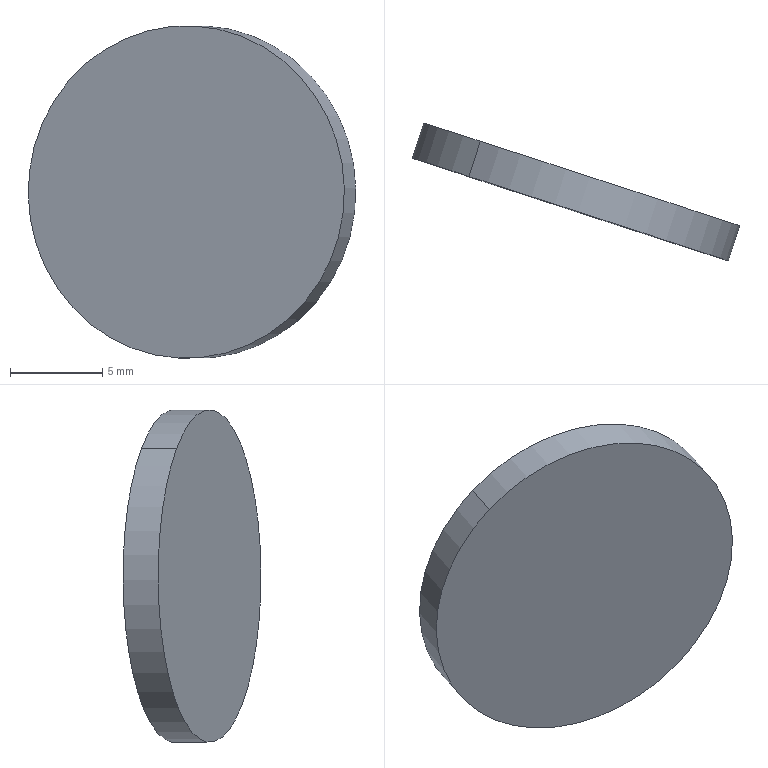Component | SolidWorks | Part3-1 | 1 solid | 4 faces | box 17.74 x 7.46 x 18 mm | volume 509 mm3 | cylinder 2 | plane 2 | commonest cylinder face diameters 18 x2
build123d program:
from build123d import *

# Parameters (mm, degrees)
SKETCH1_R           = 9
BOSS_EXTRUDE1_DEPTH = 2


with BuildPart() as part:
    # Sketch1 → Boss-Extrude1 (new body)
    with BuildSketch(Plane(origin=(0, 0, 0), x_dir=(1, 0, 0), z_dir=(0, 1, 0))):
        with Locations(Location((0, 0, 0), (0, 0, 270))):
            Circle(SKETCH1_R)
    extrude(amount=BOSS_EXTRUDE1_DEPTH)


solid = part.part

# Placed as in the assembly
solid = solid.moved(Location((-115.372, -67.891, 1043.05), (-1.302, -4.002, 161.954)))
STEP:
#1=CARTESIAN_POINT('',(-4.758,-2.603,41.337));
#2=VERTEX_POINT('',#1);
#3=CARTESIAN_POINT('',(-4.326,-2.743,40.793));
#4=VERTEX_POINT('',#3);
#5=CARTESIAN_POINT('',(-4.542,-2.673,41.065));
#6=DIRECTION('',(0.309,0.9511,-0.));
#7=DIRECTION('',(-0.6103,0.1983,0.767));
#8=AXIS2_PLACEMENT_3D('',#5,#6,#7);
#9=CIRCLE('',#8,0.3543);
#10=EDGE_CURVE('',#2,#4,#9,.T.);
#11=ORIENTED_EDGE('',*,*,#10,.F.);
#12=CARTESIAN_POINT('',(-4.783,-2.678,41.337));
#13=VERTEX_POINT('',#12);
#14=CARTESIAN_POINT('',(-4.758,-2.603,41.337));
#15=DIRECTION('',(-0.309,-0.9511,0.));
#16=VECTOR('',#15,39.37);
#17=LINE('',#14,#16);
#18=EDGE_CURVE('',#2,#13,#17,.T.);
#19=ORIENTED_EDGE('',*,*,#18,.T.);
#20=CARTESIAN_POINT('',(-4.35,-2.818,40.793));
#21=VERTEX_POINT('',#20);
#22=CARTESIAN_POINT('',(-4.567,-2.748,41.065));
#23=DIRECTION('',(0.309,0.9511,-0.));
#24=DIRECTION('',(-0.6103,0.1983,0.767));
#25=AXIS2_PLACEMENT_3D('',#22,#23,#24);
#26=CIRCLE('',#25,0.3543);
#27=EDGE_CURVE('',#13,#21,#26,.T.);
#28=ORIENTED_EDGE('',*,*,#27,.T.);
#29=CARTESIAN_POINT('',(-4.326,-2.743,40.793));
#30=DIRECTION('',(-0.309,-0.9511,0.));
#31=VECTOR('',#30,39.37);
#32=LINE('',#29,#31);
#33=EDGE_CURVE('',#4,#21,#32,.T.);
#34=ORIENTED_EDGE('',*,*,#33,.F.);
#35=EDGE_LOOP('',(#11,#19,#28,#34));
#36=FACE_OUTER_BOUND('',#35,.T.);
#37=CARTESIAN_POINT('',(-4.542,-2.673,41.065));
#38=DIRECTION('',(-0.309,-0.9511,0.));
#39=DIRECTION('',(0.6103,-0.1983,-0.767));
#40=AXIS2_PLACEMENT_3D('',#37,#38,#39);
#41=CYLINDRICAL_SURFACE('',#40,0.3543);
#42=ADVANCED_FACE('',(#36),#41,.T.);
#43=ORIENTED_EDGE('',*,*,#18,.F.);
#44=CARTESIAN_POINT('',(-4.542,-2.673,41.065));
#45=DIRECTION('',(0.309,0.9511,-0.));
#46=DIRECTION('',(-0.6103,0.1983,0.767));
#47=AXIS2_PLACEMENT_3D('',#44,#45,#46);
#48=CIRCLE('',#47,0.3543);
#49=EDGE_CURVE('',#4,#2,#48,.T.);
#50=ORIENTED_EDGE('',*,*,#49,.F.);
#51=ORIENTED_EDGE('',*,*,#33,.T.);
#52=CARTESIAN_POINT('',(-4.567,-2.748,41.065));
#53=DIRECTION('',(0.309,0.9511,-0.));
#54=DIRECTION('',(-0.6103,0.1983,0.767));
#55=AXIS2_PLACEMENT_3D('',#52,#53,#54);
#56=CIRCLE('',#55,0.3543);
#57=EDGE_CURVE('',#21,#13,#56,.T.);
#58=ORIENTED_EDGE('',*,*,#57,.T.);
#59=EDGE_LOOP('',(#43,#50,#51,#58));
#60=FACE_OUTER_BOUND('',#59,.T.);
#61=CARTESIAN_POINT('',(-4.542,-2.673,41.065));
#62=DIRECTION('',(-0.309,-0.9511,0.));
#63=DIRECTION('',(0.6103,-0.1983,-0.767));
#64=AXIS2_PLACEMENT_3D('',#61,#62,#63);
#65=CYLINDRICAL_SURFACE('',#64,0.3543);
#66=ADVANCED_FACE('',(#60),#65,.T.);
#67=ORIENTED_EDGE('',*,*,#49,.T.);
#68=ORIENTED_EDGE('',*,*,#10,.T.);
#69=EDGE_LOOP('',(#67,#68));
#70=FACE_OUTER_BOUND('',#69,.T.);
#71=CARTESIAN_POINT('',(-4.542,-2.673,41.065));
#72=DIRECTION('',(0.309,0.9511,-0.));
#73=DIRECTION('',(-0.6103,0.1983,0.767));
#74=AXIS2_PLACEMENT_3D('',#71,#72,#73);
#75=PLANE('',#74);
#76=ADVANCED_FACE('',(#70),#75,.T.);
#77=ORIENTED_EDGE('',*,*,#57,.F.);
#78=ORIENTED_EDGE('',*,*,#27,.F.);
#79=EDGE_LOOP('',(#77,#78));
#80=FACE_OUTER_BOUND('',#79,.T.);
#81=CARTESIAN_POINT('',(-4.567,-2.748,41.065));
#82=DIRECTION('',(0.309,0.9511,-0.));
#83=DIRECTION('',(-0.6103,0.1983,0.767));
#84=AXIS2_PLACEMENT_3D('',#81,#82,#83);
#85=PLANE('',#84);
#86=ADVANCED_FACE('',(#80),#85,.F.);
#87=CLOSED_SHELL('',(#42,#66,#76,#86));
#88=MANIFOLD_SOLID_BREP('',#87);
#89=CARTESIAN_POINT('',(0.,0.,0.));
#90=DIRECTION('',(0.,0.,1.));
#91=DIRECTION('',(1.,0.,0.));
#92=AXIS2_PLACEMENT_3D('',#89,#90,#91);
#93=(LENGTH_UNIT()NAMED_UNIT(*)SI_UNIT($,.METRE.));
#94=LENGTH_MEASURE_WITH_UNIT(LENGTH_MEASURE(0.0254),#93);
#95=DIMENSIONAL_EXPONENTS(1.,0.,0.,0.,0.,0.,0.);
#96=(CONVERSION_BASED_UNIT('',#94)LENGTH_UNIT()NAMED_UNIT(#95));
#97=UNCERTAINTY_MEASURE_WITH_UNIT(LENGTH_MEASURE(0.00001),#96,'','');
#98=(NAMED_UNIT(*)PLANE_ANGLE_UNIT()SI_UNIT($,.RADIAN.));
#99=(NAMED_UNIT(*)SI_UNIT($,.STERADIAN.)SOLID_ANGLE_UNIT());
#100=(GEOMETRIC_REPRESENTATION_CONTEXT(3)GLOBAL_UNCERTAINTY_ASSIGNED_CONTEXT((#97))GLOBAL_UNIT_ASSIGNED_CONTEXT((#96,#98,#99))REPRESENTATION_CONTEXT('',''));
#101=ADVANCED_BREP_SHAPE_REPRESENTATION('',(#88,#92),#100);
#102=COLOUR_RGB('',0.7922,0.8196,0.9333);
#103=FILL_AREA_STYLE_COLOUR('',#102);
#104=FILL_AREA_STYLE('',(#103));
#105=SURFACE_STYLE_FILL_AREA(#104);
#106=SURFACE_SIDE_STYLE('',(#105));
#107=SURFACE_STYLE_USAGE(.BOTH.,#106);
#108=PRESENTATION_STYLE_ASSIGNMENT((#107));
#109=STYLED_ITEM('',(#108),#88);
#110=(LENGTH_UNIT()NAMED_UNIT(*)SI_UNIT($,.METRE.));
#111=LENGTH_MEASURE_WITH_UNIT(LENGTH_MEASURE(0.0254),#110);
#112=DIMENSIONAL_EXPONENTS(1.,0.,0.,0.,0.,0.,0.);
#113=(CONVERSION_BASED_UNIT('',#111)LENGTH_UNIT()NAMED_UNIT(#112));
#114=UNCERTAINTY_MEASURE_WITH_UNIT(LENGTH_MEASURE(0.00001),#113,'','');
#115=(NAMED_UNIT(*)PLANE_ANGLE_UNIT()SI_UNIT($,.RADIAN.));
#116=(NAMED_UNIT(*)SI_UNIT($,.STERADIAN.)SOLID_ANGLE_UNIT());
#117=(GEOMETRIC_REPRESENTATION_CONTEXT(3)GLOBAL_UNCERTAINTY_ASSIGNED_CONTEXT((#114))GLOBAL_UNIT_ASSIGNED_CONTEXT((#113,#115,#116))REPRESENTATION_CONTEXT('',''));
#118=MECHANICAL_DESIGN_GEOMETRIC_PRESENTATION_REPRESENTATION('',(#109),#117);
#119=PRESENTATION_LAYER_ASSIGNMENT('','',(#109));